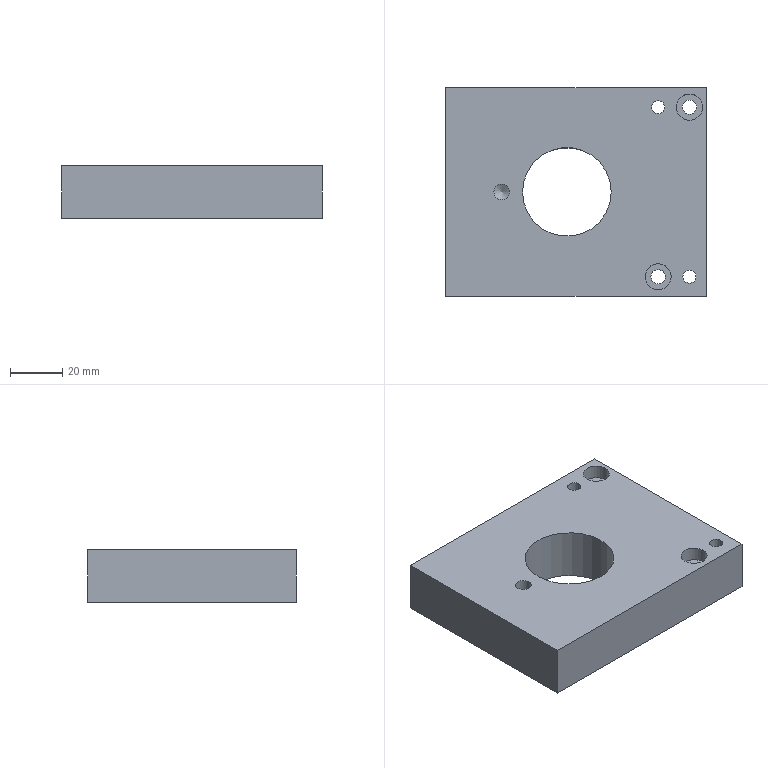Component | NX | DRILL_JIG_PLATE | 1 solid | 17 faces | volume 139082 mm3 | plane 8 | cylinder 8 | cone 1 | commonest cylinder face diameters 5.5 x2 10 x2 5 x2 34 x1 6 x1